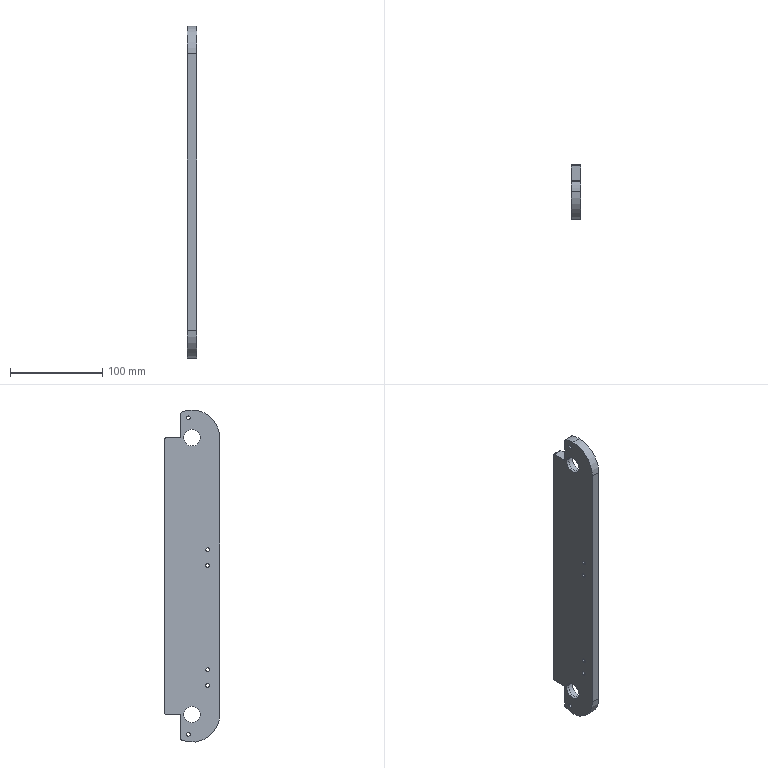Component | SolidWorks | ZHDJ-G006-1 | 1 solid | 37 faces | volume 193462 mm3 | cylinder 27 | plane 10 | commonest cylinder face diameters 4 x8 4.2 x8 22 x4 18 x4 60 x3